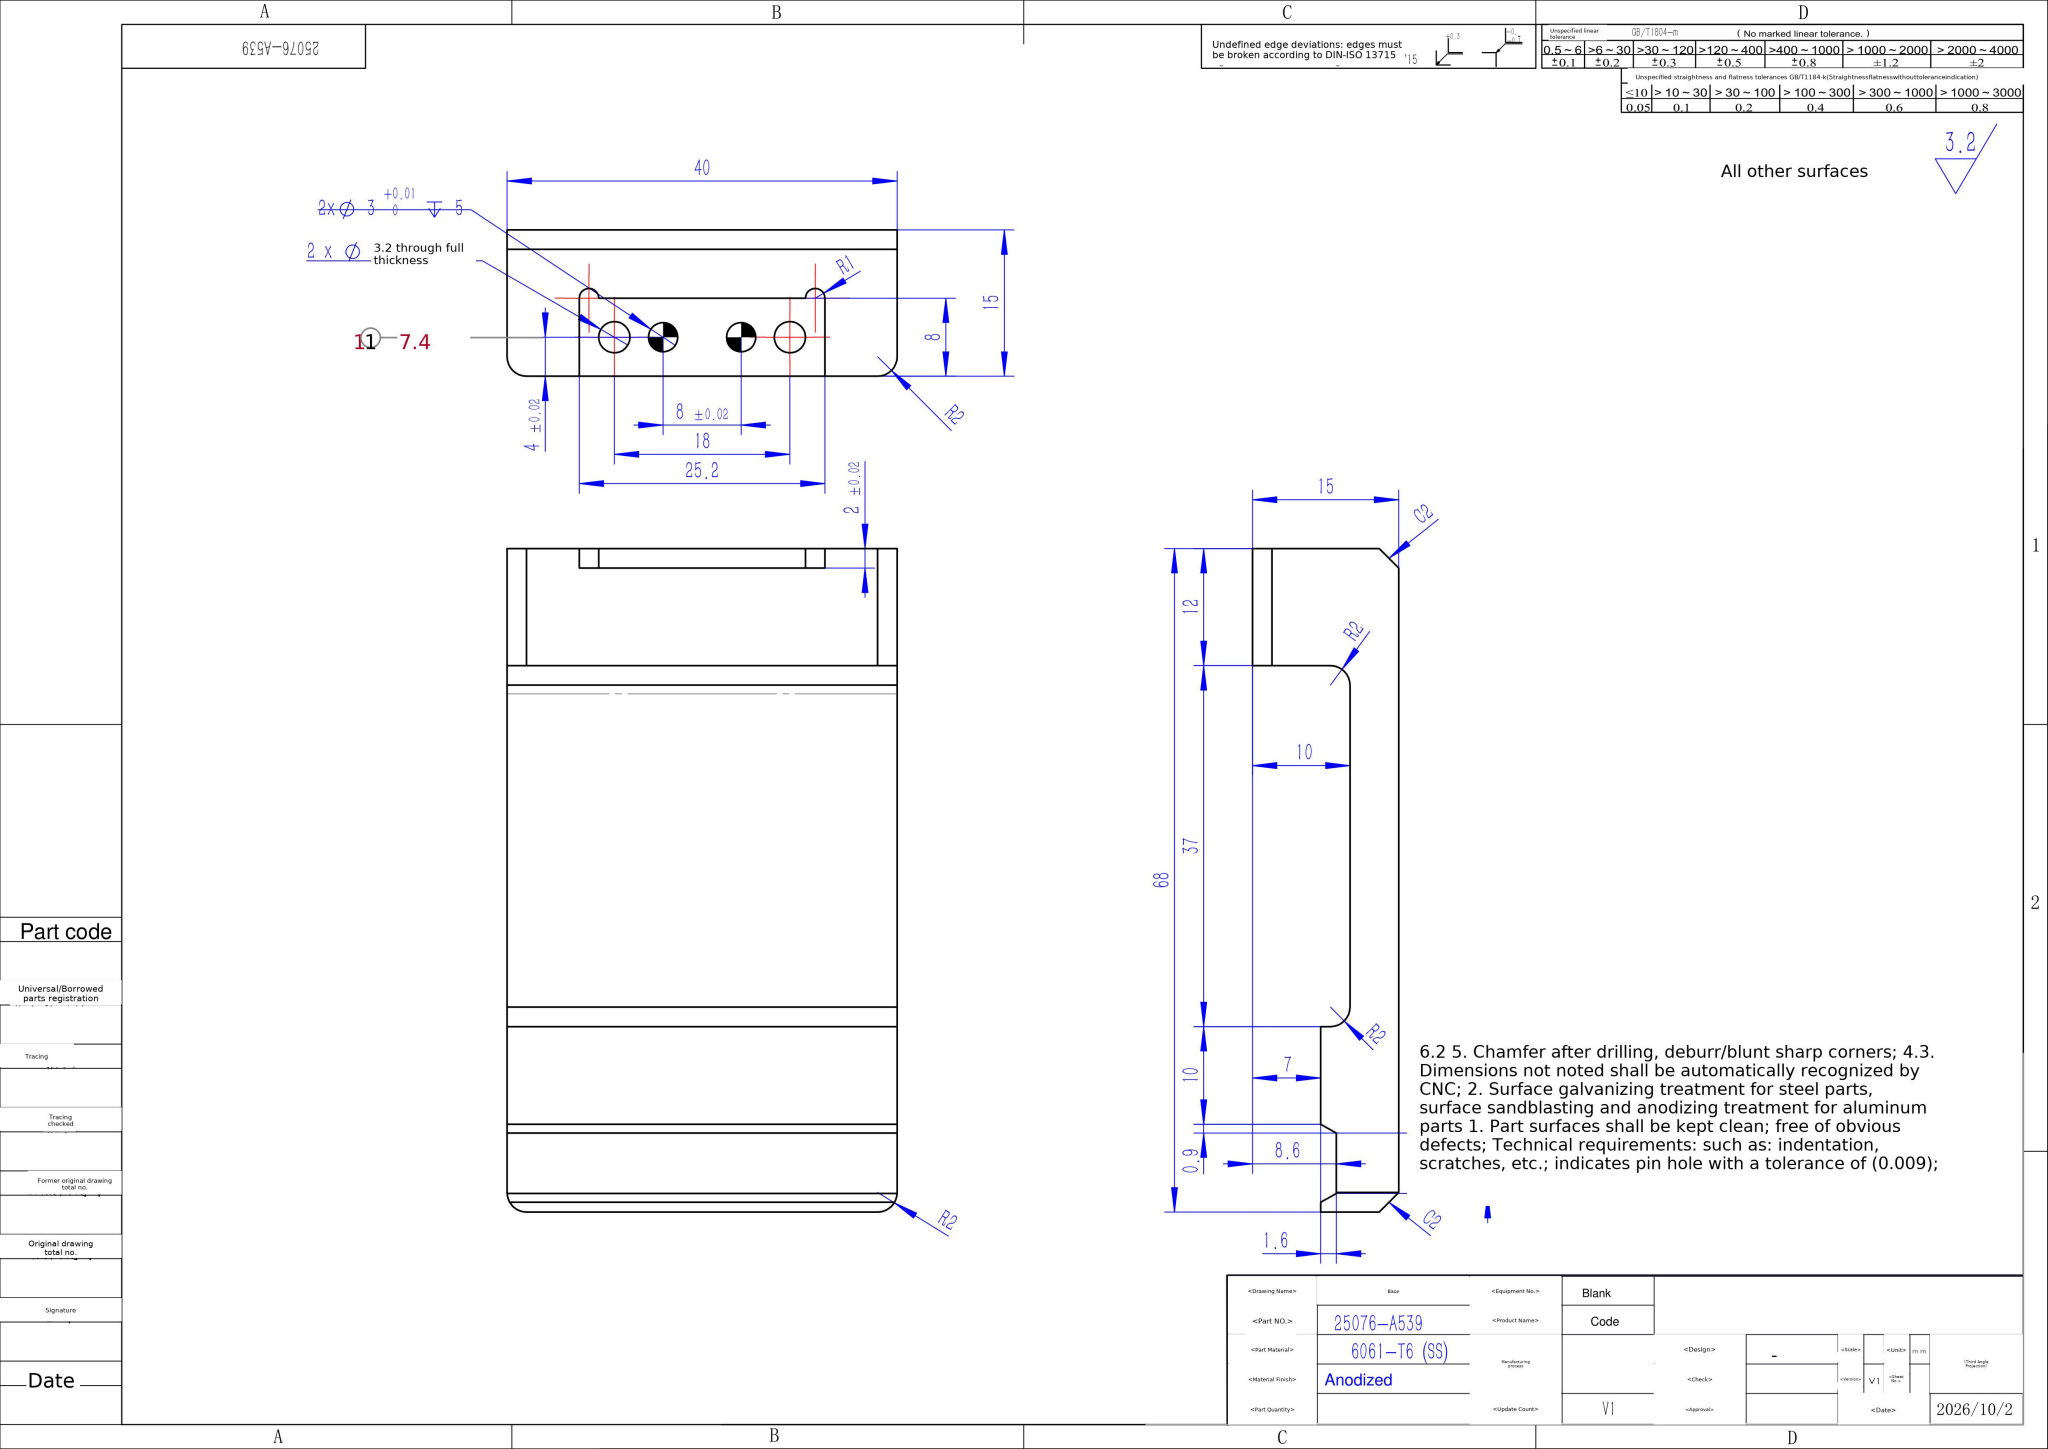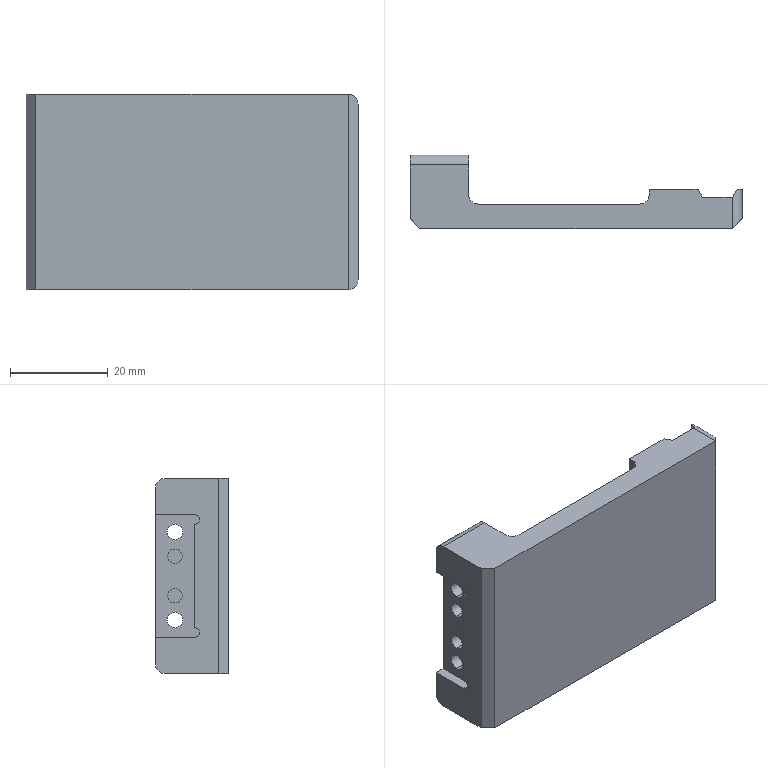Part | SolidWorks | mm | material 6061-T6 (SS) | 1 solid | 38 faces | box 68 x 15 x 40 mm | volume 19462 mm3 | plane 22 | cylinder 16 | commonest cylinder face diameters 4 x6 3 x4 3.2 x4 2 x2